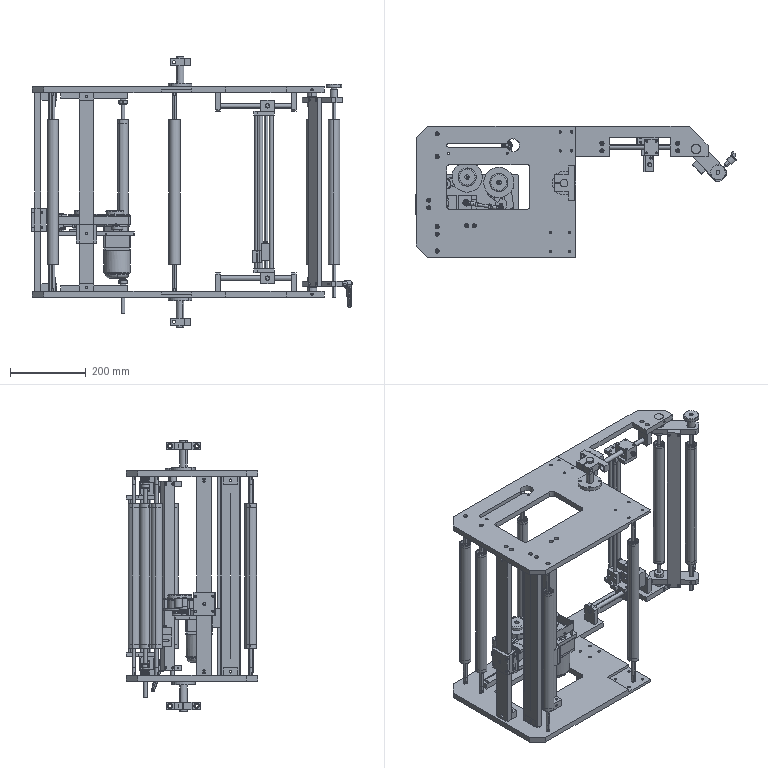Assembly | SolidWorks | mm | 66 component files | 98 solids | 4055 faces | box 845.04 x 346 x 715 mm | volume 8463848 mm3 | plane 2324 | cylinder 1250 | cone 368 | torus 105 | sphere 8 | commonest cylinder face diameters 0.4 x172 5 x130 6 x117 10 x87 7 x74 4.2 x68 20 x55 11 x54
Bill of materials:
AdjustingScrew | 1 |  | Revolved stepped cylindrical part: wide, short disc-shaped head on a narrower cylindrical shank, with a short reduced-diameter neck between them. A through or blind axial bore runs down the center and a small radial hole goes through the side of the head.
CodingMachine | 1 |  | Multi-body mechanism assembly: a rectangular base plate with two large stepped round wheel/pulley-like bodies on top, smaller rollers and a curved belt-like loop at one end, a linkage rod with ball-end joints, a frame of thin vertical posts and an upper rail, a cylindrical housing with a rounded end cap hanging below the plate, and a rectangular box with a rectangular opening on one edge.
CodingMachineSupport | 1 |  | Long, slender rectangular bar/flat strip with one small hole near each end, running through the thin direction.
ConnectingBase | 2 |  | Flanged post: a round flat flange with four small through holes on a bolt circle, and a long solid cylindrical post rising from the flange center.
ConnectingPlate | 1 |  | Thin, elongated strip or bar with a lengthwise step or groove line along one face and small holes near both ends.
Cover | 1 |  | Square flat plate with a thickness that is substantial for its size. It has four through holes near the corners and one through hole at the center.
FilmConnectionPlate | 1 |  | Long C-shaped (U-channel) bent profile with rounded bend corners. The web has a small hole near each end and a thin longitudinal line or slot.
FilmGuideRodAxis | 1 |  | Long, thin solid round rod/pin with a faceted circular cross-section. Faint circumferential lines appear near both ends.
FixedSeat | 2 |  | T-shaped block: a wider body with a large through bore, split by a narrow slot from one side into the bore. A crossbar base has two through holes, one at each end, perpendicular to the bore.
Gear | 2 |  | Hub-and-gear part: a straight-toothed spur gear section on one end, a reduced-diameter neck, and a plain cylindrical hub on the other end. The hub has a central bore with a counterbore and a radial hole through its side.
LargeSidePlate(1) | 1 |  | Large flat plate with two chamfered corners on one side. It has a large rounded-corner rectangular cutout, a long narrow slot that ends in a larger round hole, and many small through holes in pairs and groups. Shallow steps or notches appear along the underside edges.
LargeSidePlate(2) | 1 |  | Large flat plate with nearly the same outline and hole pattern as the companion plate: chamfered corners, a rounded rectangular window, and a slot ending in a round hole. It differs by a square region at one corner bounded by visible edges, and an edge step or notch along one side.
LeftSupportBlock | 1 |  | Flat elongated plate with chamfered corners at both ends and two large through holes near the ends; small cross holes enter one long edge face.
LongGearAxis | 1 |  | Long, slender solid cylindrical rod with chamfered or beveled end edges.
M5AdjustableHandle | 1 |  | L-shaped lever-like body: a cylindrical hub with a tapered, slightly curved arm projecting from it, plus a stepped axial stud with a hexagonal section and a smaller cylindrical pin end.
NameDuplicate-1Crossbar | 1 |  | Long, thin rectangular bar or strip with one small hole near each end, passing through the narrow face.
NameDuplicate-1SupportBlock | 6 |  | Rectangular block with two parallel through holes from the top face and one perpendicular through hole across the side face.
PhotoelectricBracket | 1 |  | Flat bar bracket with a long slot and two round holes, joined at one end to a taller block that has a vertical bore and a slit cut fully through it.
PhotoelectricSensor | 1 |  | Rectangular housing-like body with an angled lower front face, a knurled cylindrical knob on one end, a short round boss and a small pin on top, and two side through holes near the base.
PhotoelectricSlideRod | 2 |  | Long rectangular bar with a row of small, regularly spaced teeth along one long edge and an oblong slot near each end.
Rack | 2 |  | Flat elongated plate with chamfered corners at both ends, one large and one small through hole, and several small cross holes in the edge faces.
RightSupportBlock | 1 |  | Long, thin-walled cylindrical tube with a plain uniform outer diameter.
Roller1 | 6 |  | Plain solid cylindrical rod or pin with small chamfers at both ends.
RollerAxis1 | 4 |  | Very long, slender cylindrical rod with faint circumferential lines near both ends and a conical feature on the end face.
Roller1-1 | 1 |  | Long straight round tube of constant diameter with a concentric through bore (annular cross-section) and flat square-cut ends.
RollerAxis3 | 1 |  | Long slender solid round rod of constant diameter with flat ends.
RubberHolder | 1 |  | Rectangular block with a rectangular channel cut through it, giving a U-shaped (channel) cross-section. Two round holes are in one outer face.
RubberPlate | 1 |  | Thin flat square plate of uniform thickness with no holes or cutouts.
RubberPlateBaffle | 2 |  | Equal-thickness L-shaped angle bracket with legs of unequal width. Two round through holes are in the narrower leg.
SCLinearBearing | 2 |  | Rectangular block with a large cylindrical through bore across one pair of faces. Four small holes are near the corners of the top face, and a smaller round hole is centered on an adjacent face.
SidePlate(1) | 1 |  | Long flat plate with a large rectangular notch cut into one long edge and one chamfered corner. One end region is thinner (a stepped thickness). It has several small holes, one larger round hole near the chamfered end, and a small hole in the end edge face.
SidePlate(2) | 1 |  | Long flat plate with the same outline as unnamed part: a rectangular edge notch, a chamfered corner, small hole pairs and a larger round hole. The thinner end section is stepped on the opposite face, so the top surface is flush.
SmallHandwheel | 2 |  | Headed cylindrical pin: a short large-diameter round head on a smaller-diameter plain cylindrical shank. The outer head face is slightly domed.
SmoothRod | 4 |  | Long slender small-diameter tube with a small concentric bore of constant outer diameter.
SupportAxis | 2 |  | Solid round cylinder with flat ends and one narrow circumferential groove part-way along its length.
SupportBase | 4 |  | Thick rectangular block with two chamfered top corners on its main face. A large round through hole is in the upper part of the main face, and a small round hole is in the top face and/or a narrow face.
SupportPlate | 2 |  | Flat plate of constant thickness. Its outline is a rectangle with one smaller rectangular tab sticking out from the middle of one long edge. It has eight plain round holes that go all the way through. The holes are all about the same size.
Mates:
1. coincident | PhotoelectricBracket-1 face at (185.293, 491.5, -185.544) dir (0, -1, 0) | PhotoelectricSensor-1 face at (207.293, 491.5, -181.003) dir (0, -1, 0)
2. coincident | PhotoelectricBracket-1 face at (185.293, 586.5, -185.544) dir (1, 0, 0) | PhotoelectricSensor-1 face at (185.293, 491.5, -181.003) dir (-1, 0, 0)